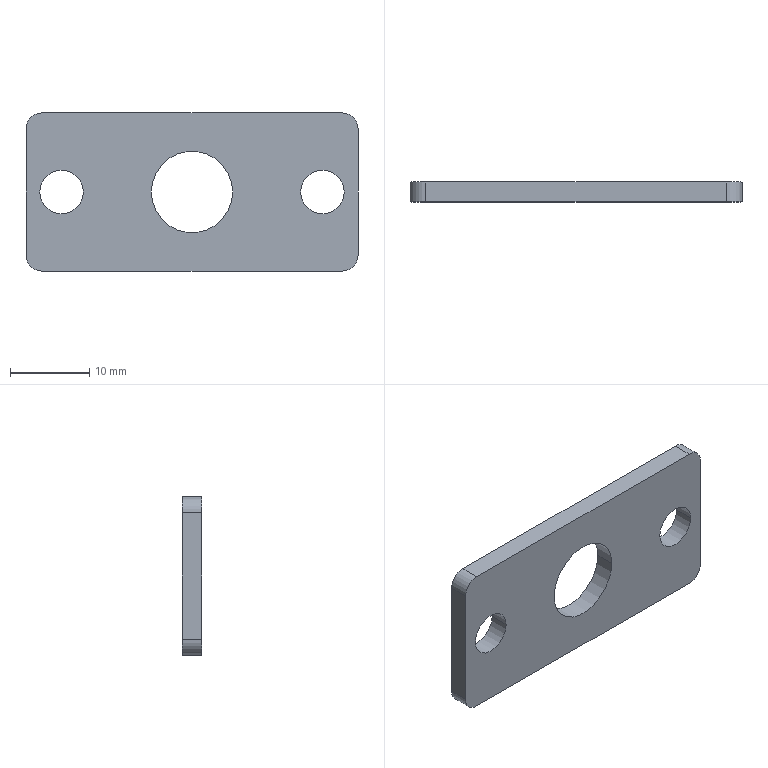Component | SolidWorks | PB_16x75_S_U_FA_M_2_0-1_F_PB12FA_16-1 | 1 solid | 16 faces | box 42 x 2.5 x 20 mm | volume 1764 mm3 | cylinder 10 | plane 6 | commonest cylinder face diameters 5.5 x4 4 x4 10.3 x2
build123d program:
from build123d import *

# Parameters (mm, degrees)
SKETCH1_R      = 2.75
SKETCH1_R_2    = 5.15
EXTRUDE1_DEPTH = 2.5


with BuildPart() as part:
    # Sketch1 → Extrude1 (new body)
    with BuildSketch(Plane.XY):
        with BuildLine():
            Line((-21, 8), (-21, -8))
            ThreePointArc((-21, -8), (-20.414, -9.414), (-19, -10))
            Line((-19, -10), (19, -10))
            ThreePointArc((19, -10), (20.414, -9.414), (21, -8))
            Line((21, -8), (21, 8))
            ThreePointArc((21, 8), (20.414, 9.414), (19, 10))
            Line((19, 10), (-19, 10))
            ThreePointArc((-19, 10), (-20.414, 9.414), (-21, 8))
        make_face()
        with Locations((16.5, 0)):
            Circle(SKETCH1_R, mode=Mode.SUBTRACT)
        Circle(SKETCH1_R_2, mode=Mode.SUBTRACT)
        with Locations((-16.5, 0)):
            Circle(SKETCH1_R, mode=Mode.SUBTRACT)
    extrude(amount=-EXTRUDE1_DEPTH)


solid = part.part

# Placed as in the assembly
solid = solid.moved(Location((45, -225, 55), (90, 0, 0)))
STEP:
#1=COLOUR_RGB('',0.7922,0.8196,0.9333);
#2=FILL_AREA_STYLE_COLOUR('',#1);
#3=FILL_AREA_STYLE('',(#2));
#4=SURFACE_STYLE_FILL_AREA(#3);
#5=SURFACE_SIDE_STYLE('',(#4));
#6=SURFACE_STYLE_USAGE(.BOTH.,#5);
#7=PRESENTATION_STYLE_ASSIGNMENT((#6));
#8=CARTESIAN_POINT('',(1.014,-8.76,2.165));
#9=VERTEX_POINT('',#8);
#10=CARTESIAN_POINT('',(1.23,-8.76,2.165));
#11=VERTEX_POINT('',#10);
#12=CARTESIAN_POINT('',(1.122,-8.76,2.165));
#13=DIRECTION('',(0.,-1.,0.));
#14=DIRECTION('',(1.,0.,0.));
#15=AXIS2_PLACEMENT_3D('',#12,#13,#14);
#16=CIRCLE('',#15,0.1083);
#17=EDGE_CURVE('',#9,#11,#16,.T.);
#18=ORIENTED_EDGE('',*,*,#17,.F.);
#19=CARTESIAN_POINT('',(1.014,-8.858,2.165));
#20=VERTEX_POINT('',#19);
#21=CARTESIAN_POINT('',(1.014,-8.76,2.165));
#22=DIRECTION('',(0.,-1.,0.));
#23=VECTOR('',#22,39.37);
#24=LINE('',#21,#23);
#25=EDGE_CURVE('',#9,#20,#24,.T.);
#26=ORIENTED_EDGE('',*,*,#25,.T.);
#27=CARTESIAN_POINT('',(1.23,-8.858,2.165));
#28=VERTEX_POINT('',#27);
#29=CARTESIAN_POINT('',(1.122,-8.858,2.165));
#30=DIRECTION('',(0.,-1.,0.));
#31=DIRECTION('',(1.,0.,0.));
#32=AXIS2_PLACEMENT_3D('',#29,#30,#31);
#33=CIRCLE('',#32,0.1083);
#34=EDGE_CURVE('',#20,#28,#33,.T.);
#35=ORIENTED_EDGE('',*,*,#34,.T.);
#36=CARTESIAN_POINT('',(1.23,-8.76,2.165));
#37=DIRECTION('',(0.,-1.,0.));
#38=VECTOR('',#37,39.37);
#39=LINE('',#36,#38);
#40=EDGE_CURVE('',#11,#28,#39,.T.);
#41=ORIENTED_EDGE('',*,*,#40,.F.);
#42=EDGE_LOOP('',(#18,#26,#35,#41));
#43=FACE_OUTER_BOUND('',#42,.T.);
#44=CARTESIAN_POINT('',(1.122,-8.76,2.165));
#45=DIRECTION('',(0.,-1.,0.));
#46=DIRECTION('',(1.,0.,0.));
#47=AXIS2_PLACEMENT_3D('',#44,#45,#46);
#48=CYLINDRICAL_SURFACE('',#47,0.1083);
#49=ADVANCED_FACE('',(#43),#48,.F.);
#50=CARTESIAN_POINT('',(1.569,-8.76,2.165));
#51=VERTEX_POINT('',#50);
#52=CARTESIAN_POINT('',(1.974,-8.76,2.165));
#53=VERTEX_POINT('',#52);
#54=CARTESIAN_POINT('',(1.772,-8.76,2.165));
#55=DIRECTION('',(0.,-1.,0.));
#56=DIRECTION('',(1.,0.,0.));
#57=AXIS2_PLACEMENT_3D('',#54,#55,#56);
#58=CIRCLE('',#57,0.2028);
#59=EDGE_CURVE('',#51,#53,#58,.T.);
#60=ORIENTED_EDGE('',*,*,#59,.F.);
#61=CARTESIAN_POINT('',(1.569,-8.858,2.165));
#62=VERTEX_POINT('',#61);
#63=CARTESIAN_POINT('',(1.569,-8.76,2.165));
#64=DIRECTION('',(0.,-1.,0.));
#65=VECTOR('',#64,39.37);
#66=LINE('',#63,#65);
#67=EDGE_CURVE('',#51,#62,#66,.T.);
#68=ORIENTED_EDGE('',*,*,#67,.T.);
#69=CARTESIAN_POINT('',(1.974,-8.858,2.165));
#70=VERTEX_POINT('',#69);
#71=CARTESIAN_POINT('',(1.772,-8.858,2.165));
#72=DIRECTION('',(0.,-1.,0.));
#73=DIRECTION('',(1.,0.,0.));
#74=AXIS2_PLACEMENT_3D('',#71,#72,#73);
#75=CIRCLE('',#74,0.2028);
#76=EDGE_CURVE('',#62,#70,#75,.T.);
#77=ORIENTED_EDGE('',*,*,#76,.T.);
#78=CARTESIAN_POINT('',(1.974,-8.76,2.165));
#79=DIRECTION('',(0.,-1.,0.));
#80=VECTOR('',#79,39.37);
#81=LINE('',#78,#80);
#82=EDGE_CURVE('',#53,#70,#81,.T.);
#83=ORIENTED_EDGE('',*,*,#82,.F.);
#84=EDGE_LOOP('',(#60,#68,#77,#83));
#85=FACE_OUTER_BOUND('',#84,.T.);
#86=CARTESIAN_POINT('',(1.772,-8.76,2.165));
#87=DIRECTION('',(0.,-1.,0.));
#88=DIRECTION('',(1.,0.,0.));
#89=AXIS2_PLACEMENT_3D('',#86,#87,#88);
#90=CYLINDRICAL_SURFACE('',#89,0.2028);
#91=ADVANCED_FACE('',(#85),#90,.F.);
#92=CARTESIAN_POINT('',(2.313,-8.76,2.165));
#93=VERTEX_POINT('',#92);
#94=CARTESIAN_POINT('',(2.53,-8.76,2.165));
#95=VERTEX_POINT('',#94);
#96=CARTESIAN_POINT('',(2.421,-8.76,2.165));
#97=DIRECTION('',(0.,-1.,0.));
#98=DIRECTION('',(1.,0.,0.));
#99=AXIS2_PLACEMENT_3D('',#96,#97,#98);
#100=CIRCLE('',#99,0.1083);
#101=EDGE_CURVE('',#93,#95,#100,.T.);
#102=ORIENTED_EDGE('',*,*,#101,.F.);
#103=CARTESIAN_POINT('',(2.313,-8.858,2.165));
#104=VERTEX_POINT('',#103);
#105=CARTESIAN_POINT('',(2.313,-8.76,2.165));
#106=DIRECTION('',(0.,-1.,0.));
#107=VECTOR('',#106,39.37);
#108=LINE('',#105,#107);
#109=EDGE_CURVE('',#93,#104,#108,.T.);
#110=ORIENTED_EDGE('',*,*,#109,.T.);
#111=CARTESIAN_POINT('',(2.53,-8.858,2.165));
#112=VERTEX_POINT('',#111);
#113=CARTESIAN_POINT('',(2.421,-8.858,2.165));
#114=DIRECTION('',(0.,-1.,0.));
#115=DIRECTION('',(1.,0.,0.));
#116=AXIS2_PLACEMENT_3D('',#113,#114,#115);
#117=CIRCLE('',#116,0.1083);
#118=EDGE_CURVE('',#104,#112,#117,.T.);
#119=ORIENTED_EDGE('',*,*,#118,.T.);
#120=CARTESIAN_POINT('',(2.53,-8.76,2.165));
#121=DIRECTION('',(0.,-1.,0.));
#122=VECTOR('',#121,39.37);
#123=LINE('',#120,#122);
#124=EDGE_CURVE('',#95,#112,#123,.T.);
#125=ORIENTED_EDGE('',*,*,#124,.F.);
#126=EDGE_LOOP('',(#102,#110,#119,#125));
#127=FACE_OUTER_BOUND('',#126,.T.);
#128=CARTESIAN_POINT('',(2.421,-8.76,2.165));
#129=DIRECTION('',(0.,-1.,0.));
#130=DIRECTION('',(1.,0.,0.));
#131=AXIS2_PLACEMENT_3D('',#128,#129,#130);
#132=CYLINDRICAL_SURFACE('',#131,0.1083);
#133=ADVANCED_FACE('',(#127),#132,.F.);
#134=CARTESIAN_POINT('',(1.024,-8.858,2.559));
#135=VERTEX_POINT('',#134);
#136=CARTESIAN_POINT('',(0.9449,-8.858,2.48));
#137=VERTEX_POINT('',#136);
#138=CARTESIAN_POINT('',(1.024,-8.858,2.48));
#139=DIRECTION('',(0.,-1.,0.));
#140=DIRECTION('',(1.,0.,0.));
#141=AXIS2_PLACEMENT_3D('',#138,#139,#140);
#142=CIRCLE('',#141,0.07874);
#143=EDGE_CURVE('',#135,#137,#142,.T.);
#144=ORIENTED_EDGE('',*,*,#143,.F.);
#145=CARTESIAN_POINT('',(1.024,-8.76,2.559));
#146=VERTEX_POINT('',#145);
#147=CARTESIAN_POINT('',(1.024,-8.76,2.559));
#148=DIRECTION('',(0.,-1.,0.));
#149=VECTOR('',#148,39.37);
#150=LINE('',#147,#149);
#151=EDGE_CURVE('',#146,#135,#150,.T.);
#152=ORIENTED_EDGE('',*,*,#151,.F.);
#153=CARTESIAN_POINT('',(0.9449,-8.76,2.48));
#154=VERTEX_POINT('',#153);
#155=CARTESIAN_POINT('',(1.024,-8.76,2.48));
#156=DIRECTION('',(0.,-1.,0.));
#157=DIRECTION('',(1.,0.,0.));
#158=AXIS2_PLACEMENT_3D('',#155,#156,#157);
#159=CIRCLE('',#158,0.07874);
#160=EDGE_CURVE('',#146,#154,#159,.T.);
#161=ORIENTED_EDGE('',*,*,#160,.T.);
#162=CARTESIAN_POINT('',(0.9449,-8.76,2.48));
#163=DIRECTION('',(0.,-1.,0.));
#164=VECTOR('',#163,39.37);
#165=LINE('',#162,#164);
#166=EDGE_CURVE('',#154,#137,#165,.T.);
#167=ORIENTED_EDGE('',*,*,#166,.T.);
#168=EDGE_LOOP('',(#144,#152,#161,#167));
#169=FACE_OUTER_BOUND('',#168,.T.);
#170=CARTESIAN_POINT('',(1.024,-8.76,2.48));
#171=DIRECTION('',(0.,-1.,0.));
#172=DIRECTION('',(1.,0.,0.));
#173=AXIS2_PLACEMENT_3D('',#170,#171,#172);
#174=CYLINDRICAL_SURFACE('',#173,0.07874);
#175=ADVANCED_FACE('',(#169),#174,.T.);
#176=CARTESIAN_POINT('',(2.52,-8.858,2.559));
#177=VERTEX_POINT('',#176);
#178=CARTESIAN_POINT('',(2.52,-8.858,2.559));
#179=DIRECTION('',(-1.,0.,0.));
#180=VECTOR('',#179,39.37);
#181=LINE('',#178,#180);
#182=EDGE_CURVE('',#177,#135,#181,.T.);
#183=ORIENTED_EDGE('',*,*,#182,.F.);
#184=CARTESIAN_POINT('',(2.52,-8.76,2.559));
#185=VERTEX_POINT('',#184);
#186=CARTESIAN_POINT('',(2.52,-8.76,2.559));
#187=DIRECTION('',(0.,-1.,0.));
#188=VECTOR('',#187,39.37);
#189=LINE('',#186,#188);
#190=EDGE_CURVE('',#185,#177,#189,.T.);
#191=ORIENTED_EDGE('',*,*,#190,.F.);
#192=CARTESIAN_POINT('',(2.52,-8.76,2.559));
#193=DIRECTION('',(-1.,0.,0.));
#194=VECTOR('',#193,39.37);
#195=LINE('',#192,#194);
#196=EDGE_CURVE('',#185,#146,#195,.T.);
#197=ORIENTED_EDGE('',*,*,#196,.T.);
#198=ORIENTED_EDGE('',*,*,#151,.T.);
#199=EDGE_LOOP('',(#183,#191,#197,#198));
#200=FACE_OUTER_BOUND('',#199,.T.);
#201=CARTESIAN_POINT('',(2.52,-8.76,2.559));
#202=DIRECTION('',(0.,0.,1.));
#203=DIRECTION('',(0.,-1.,0.));
#204=AXIS2_PLACEMENT_3D('',#201,#202,#203);
#205=PLANE('',#204);
#206=ADVANCED_FACE('',(#200),#205,.T.);
#207=CARTESIAN_POINT('',(2.598,-8.858,2.48));
#208=VERTEX_POINT('',#207);
#209=CARTESIAN_POINT('',(2.52,-8.858,2.48));
#210=DIRECTION('',(0.,-1.,0.));
#211=DIRECTION('',(1.,0.,0.));
#212=AXIS2_PLACEMENT_3D('',#209,#210,#211);
#213=CIRCLE('',#212,0.07874);
#214=EDGE_CURVE('',#208,#177,#213,.T.);
#215=ORIENTED_EDGE('',*,*,#214,.F.);
#216=CARTESIAN_POINT('',(2.598,-8.76,2.48));
#217=VERTEX_POINT('',#216);
#218=CARTESIAN_POINT('',(2.598,-8.76,2.48));
#219=DIRECTION('',(0.,-1.,0.));
#220=VECTOR('',#219,39.37);
#221=LINE('',#218,#220);
#222=EDGE_CURVE('',#217,#208,#221,.T.);
#223=ORIENTED_EDGE('',*,*,#222,.F.);
#224=CARTESIAN_POINT('',(2.52,-8.76,2.48));
#225=DIRECTION('',(0.,-1.,0.));
#226=DIRECTION('',(1.,0.,0.));
#227=AXIS2_PLACEMENT_3D('',#224,#225,#226);
#228=CIRCLE('',#227,0.07874);
#229=EDGE_CURVE('',#217,#185,#228,.T.);
#230=ORIENTED_EDGE('',*,*,#229,.T.);
#231=ORIENTED_EDGE('',*,*,#190,.T.);
#232=EDGE_LOOP('',(#215,#223,#230,#231));
#233=FACE_OUTER_BOUND('',#232,.T.);
#234=CARTESIAN_POINT('',(2.52,-8.76,2.48));
#235=DIRECTION('',(0.,-1.,0.));
#236=DIRECTION('',(1.,0.,0.));
#237=AXIS2_PLACEMENT_3D('',#234,#235,#236);
#238=CYLINDRICAL_SURFACE('',#237,0.07874);
#239=ADVANCED_FACE('',(#233),#238,.T.);
#240=CARTESIAN_POINT('',(2.598,-8.858,1.85));
#241=VERTEX_POINT('',#240);
#242=CARTESIAN_POINT('',(2.598,-8.858,1.85));
#243=DIRECTION('',(0.,0.,1.));
#244=VECTOR('',#243,39.37);
#245=LINE('',#242,#244);
#246=EDGE_CURVE('',#241,#208,#245,.T.);
#247=ORIENTED_EDGE('',*,*,#246,.F.);
#248=CARTESIAN_POINT('',(2.598,-8.76,1.85));
#249=VERTEX_POINT('',#248);
#250=CARTESIAN_POINT('',(2.598,-8.76,1.85));
#251=DIRECTION('',(0.,-1.,0.));
#252=VECTOR('',#251,39.37);
#253=LINE('',#250,#252);
#254=EDGE_CURVE('',#249,#241,#253,.T.);
#255=ORIENTED_EDGE('',*,*,#254,.F.);
#256=CARTESIAN_POINT('',(2.598,-8.76,1.85));
#257=DIRECTION('',(0.,0.,1.));
#258=VECTOR('',#257,39.37);
#259=LINE('',#256,#258);
#260=EDGE_CURVE('',#249,#217,#259,.T.);
#261=ORIENTED_EDGE('',*,*,#260,.T.);
#262=ORIENTED_EDGE('',*,*,#222,.T.);
#263=EDGE_LOOP('',(#247,#255,#261,#262));
#264=FACE_OUTER_BOUND('',#263,.T.);
#265=CARTESIAN_POINT('',(2.598,-8.76,1.85));
#266=DIRECTION('',(1.,0.,0.));
#267=DIRECTION('',(0.,1.,0.));
#268=AXIS2_PLACEMENT_3D('',#265,#266,#267);
#269=PLANE('',#268);
#270=ADVANCED_FACE('',(#264),#269,.T.);
#271=CARTESIAN_POINT('',(2.52,-8.858,1.772));
#272=VERTEX_POINT('',#271);
#273=CARTESIAN_POINT('',(2.52,-8.858,1.85));
#274=DIRECTION('',(0.,-1.,0.));
#275=DIRECTION('',(1.,0.,0.));
#276=AXIS2_PLACEMENT_3D('',#273,#274,#275);
#277=CIRCLE('',#276,0.07874);
#278=EDGE_CURVE('',#272,#241,#277,.T.);
#279=ORIENTED_EDGE('',*,*,#278,.F.);
#280=CARTESIAN_POINT('',(2.52,-8.76,1.772));
#281=VERTEX_POINT('',#280);
#282=CARTESIAN_POINT('',(2.52,-8.76,1.772));
#283=DIRECTION('',(0.,-1.,0.));
#284=VECTOR('',#283,39.37);
#285=LINE('',#282,#284);
#286=EDGE_CURVE('',#281,#272,#285,.T.);
#287=ORIENTED_EDGE('',*,*,#286,.F.);
#288=CARTESIAN_POINT('',(2.52,-8.76,1.85));
#289=DIRECTION('',(0.,-1.,0.));
#290=DIRECTION('',(1.,0.,0.));
#291=AXIS2_PLACEMENT_3D('',#288,#289,#290);
#292=CIRCLE('',#291,0.07874);
#293=EDGE_CURVE('',#281,#249,#292,.T.);
#294=ORIENTED_EDGE('',*,*,#293,.T.);
#295=ORIENTED_EDGE('',*,*,#254,.T.);
#296=EDGE_LOOP('',(#279,#287,#294,#295));
#297=FACE_OUTER_BOUND('',#296,.T.);
#298=CARTESIAN_POINT('',(2.52,-8.76,1.85));
#299=DIRECTION('',(0.,-1.,0.));
#300=DIRECTION('',(1.,0.,0.));
#301=AXIS2_PLACEMENT_3D('',#298,#299,#300);
#302=CYLINDRICAL_SURFACE('',#301,0.07874);
#303=ADVANCED_FACE('',(#297),#302,.T.);
#304=CARTESIAN_POINT('',(1.024,-8.858,1.772));
#305=VERTEX_POINT('',#304);
#306=CARTESIAN_POINT('',(1.024,-8.858,1.772));
#307=DIRECTION('',(1.,0.,0.));
#308=VECTOR('',#307,39.37);
#309=LINE('',#306,#308);
#310=EDGE_CURVE('',#305,#272,#309,.T.);
#311=ORIENTED_EDGE('',*,*,#310,.F.);
#312=CARTESIAN_POINT('',(1.024,-8.76,1.772));
#313=VERTEX_POINT('',#312);
#314=CARTESIAN_POINT('',(1.024,-8.76,1.772));
#315=DIRECTION('',(0.,-1.,0.));
#316=VECTOR('',#315,39.37);
#317=LINE('',#314,#316);
#318=EDGE_CURVE('',#313,#305,#317,.T.);
#319=ORIENTED_EDGE('',*,*,#318,.F.);
#320=CARTESIAN_POINT('',(1.024,-8.76,1.772));
#321=DIRECTION('',(1.,0.,0.));
#322=VECTOR('',#321,39.37);
#323=LINE('',#320,#322);
#324=EDGE_CURVE('',#313,#281,#323,.T.);
#325=ORIENTED_EDGE('',*,*,#324,.T.);
#326=ORIENTED_EDGE('',*,*,#286,.T.);
#327=EDGE_LOOP('',(#311,#319,#325,#326));
#328=FACE_OUTER_BOUND('',#327,.T.);
#329=CARTESIAN_POINT('',(1.024,-8.76,1.772));
#330=DIRECTION('',(0.,0.,-1.));
#331=DIRECTION('',(0.,1.,0.));
#332=AXIS2_PLACEMENT_3D('',#329,#330,#331);
#333=PLANE('',#332);
#334=ADVANCED_FACE('',(#328),#333,.T.);
#335=CARTESIAN_POINT('',(0.9449,-8.858,1.85));
#336=VERTEX_POINT('',#335);
#337=CARTESIAN_POINT('',(1.024,-8.858,1.85));
#338=DIRECTION('',(0.,-1.,0.));
#339=DIRECTION('',(1.,0.,0.));
#340=AXIS2_PLACEMENT_3D('',#337,#338,#339);
#341=CIRCLE('',#340,0.07874);
#342=EDGE_CURVE('',#336,#305,#341,.T.);
#343=ORIENTED_EDGE('',*,*,#342,.F.);
#344=CARTESIAN_POINT('',(0.9449,-8.76,1.85));
#345=VERTEX_POINT('',#344);
#346=CARTESIAN_POINT('',(0.9449,-8.76,1.85));
#347=DIRECTION('',(0.,-1.,0.));
#348=VECTOR('',#347,39.37);
#349=LINE('',#346,#348);
#350=EDGE_CURVE('',#345,#336,#349,.T.);
#351=ORIENTED_EDGE('',*,*,#350,.F.);
#352=CARTESIAN_POINT('',(1.024,-8.76,1.85));
#353=DIRECTION('',(0.,-1.,0.));
#354=DIRECTION('',(1.,0.,0.));
#355=AXIS2_PLACEMENT_3D('',#352,#353,#354);
#356=CIRCLE('',#355,0.07874);
#357=EDGE_CURVE('',#345,#313,#356,.T.);
#358=ORIENTED_EDGE('',*,*,#357,.T.);
#359=ORIENTED_EDGE('',*,*,#318,.T.);
#360=EDGE_LOOP('',(#343,#351,#358,#359));
#361=FACE_OUTER_BOUND('',#360,.T.);
#362=CARTESIAN_POINT('',(1.024,-8.76,1.85));
#363=DIRECTION('',(0.,-1.,0.));
#364=DIRECTION('',(1.,0.,0.));
#365=AXIS2_PLACEMENT_3D('',#362,#363,#364);
#366=CYLINDRICAL_SURFACE('',#365,0.07874);
#367=ADVANCED_FACE('',(#361),#366,.T.);
#368=CARTESIAN_POINT('',(0.9449,-8.858,2.48));
#369=DIRECTION('',(0.,0.,-1.));
#370=VECTOR('',#369,39.37);
#371=LINE('',#368,#370);
#372=EDGE_CURVE('',#137,#336,#371,.T.);
#373=ORIENTED_EDGE('',*,*,#372,.F.);
#374=ORIENTED_EDGE('',*,*,#166,.F.);
#375=CARTESIAN_POINT('',(0.9449,-8.76,2.48));
#376=DIRECTION('',(0.,0.,-1.));
#377=VECTOR('',#376,39.37);
#378=LINE('',#375,#377);
#379=EDGE_CURVE('',#154,#345,#378,.T.);
#380=ORIENTED_EDGE('',*,*,#379,.T.);
#381=ORIENTED_EDGE('',*,*,#350,.T.);
#382=EDGE_LOOP('',(#373,#374,#380,#381));
#383=FACE_OUTER_BOUND('',#382,.T.);
#384=CARTESIAN_POINT('',(0.9449,-8.76,2.48));
#385=DIRECTION('',(-1.,0.,0.));
#386=DIRECTION('',(0.,-1.,0.));
#387=AXIS2_PLACEMENT_3D('',#384,#385,#386);
#388=PLANE('',#387);
#389=ADVANCED_FACE('',(#383),#388,.T.);
#390=CARTESIAN_POINT('',(1.122,-8.76,2.165));
#391=DIRECTION('',(0.,-1.,0.));
#392=DIRECTION('',(1.,0.,0.));
#393=AXIS2_PLACEMENT_3D('',#390,#391,#392);
#394=CIRCLE('',#393,0.1083);
#395=EDGE_CURVE('',#11,#9,#394,.T.);
#396=ORIENTED_EDGE('',*,*,#395,.T.);
#397=ORIENTED_EDGE('',*,*,#17,.T.);
#398=EDGE_LOOP('',(#396,#397));
#399=FACE_BOUND('',#398,.T.);
#400=CARTESIAN_POINT('',(1.772,-8.76,2.165));
#401=DIRECTION('',(0.,-1.,0.));
#402=DIRECTION('',(1.,0.,0.));
#403=AXIS2_PLACEMENT_3D('',#400,#401,#402);
#404=CIRCLE('',#403,0.2028);
#405=EDGE_CURVE('',#53,#51,#404,.T.);
#406=ORIENTED_EDGE('',*,*,#405,.T.);
#407=ORIENTED_EDGE('',*,*,#59,.T.);
#408=EDGE_LOOP('',(#406,#407));
#409=FACE_BOUND('',#408,.T.);
#410=CARTESIAN_POINT('',(2.421,-8.76,2.165));
#411=DIRECTION('',(0.,-1.,0.));
#412=DIRECTION('',(1.,0.,0.));
#413=AXIS2_PLACEMENT_3D('',#410,#411,#412);
#414=CIRCLE('',#413,0.1083);
#415=EDGE_CURVE('',#95,#93,#414,.T.);
#416=ORIENTED_EDGE('',*,*,#415,.T.);
#417=ORIENTED_EDGE('',*,*,#101,.T.);
#418=EDGE_LOOP('',(#416,#417));
#419=FACE_BOUND('',#418,.T.);
#420=ORIENTED_EDGE('',*,*,#160,.F.);
#421=ORIENTED_EDGE('',*,*,#196,.F.);
#422=ORIENTED_EDGE('',*,*,#229,.F.);
#423=ORIENTED_EDGE('',*,*,#260,.F.);
#424=ORIENTED_EDGE('',*,*,#293,.F.);
#425=ORIENTED_EDGE('',*,*,#324,.F.);
#426=ORIENTED_EDGE('',*,*,#357,.F.);
#427=ORIENTED_EDGE('',*,*,#379,.F.);
#428=EDGE_LOOP('',(#420,#421,#422,#423,#424,#425,#426,#427));
#429=FACE_OUTER_BOUND('',#428,.T.);
#430=CARTESIAN_POINT('',(1.024,-8.76,2.48));
#431=DIRECTION('',(0.,-1.,0.));
#432=DIRECTION('',(1.,0.,0.));
#433=AXIS2_PLACEMENT_3D('',#430,#431,#432);
#434=PLANE('',#433);
#435=ADVANCED_FACE('',(#399,#409,#419,#429),#434,.F.);
#436=CARTESIAN_POINT('',(1.122,-8.858,2.165));
#437=DIRECTION('',(0.,-1.,0.));
#438=DIRECTION('',(1.,0.,0.));
#439=AXIS2_PLACEMENT_3D('',#436,#437,#438);
#440=CIRCLE('',#439,0.1083);
#441=EDGE_CURVE('',#28,#20,#440,.T.);
#442=ORIENTED_EDGE('',*,*,#441,.F.);
#443=ORIENTED_EDGE('',*,*,#34,.F.);
#444=EDGE_LOOP('',(#442,#443));
#445=FACE_BOUND('',#444,.T.);
#446=CARTESIAN_POINT('',(1.772,-8.858,2.165));
#447=DIRECTION('',(0.,-1.,0.));
#448=DIRECTION('',(1.,0.,0.));
#449=AXIS2_PLACEMENT_3D('',#446,#447,#448);
#450=CIRCLE('',#449,0.2028);
#451=EDGE_CURVE('',#70,#62,#450,.T.);
#452=ORIENTED_EDGE('',*,*,#451,.F.);
#453=ORIENTED_EDGE('',*,*,#76,.F.);
#454=EDGE_LOOP('',(#452,#453));
#455=FACE_BOUND('',#454,.T.);
#456=CARTESIAN_POINT('',(2.421,-8.858,2.165));
#457=DIRECTION('',(0.,-1.,0.));
#458=DIRECTION('',(1.,0.,0.));
#459=AXIS2_PLACEMENT_3D('',#456,#457,#458);
#460=CIRCLE('',#459,0.1083);
#461=EDGE_CURVE('',#112,#104,#460,.T.);
#462=ORIENTED_EDGE('',*,*,#461,.F.);
#463=ORIENTED_EDGE('',*,*,#118,.F.);
#464=EDGE_LOOP('',(#462,#463));
#465=FACE_BOUND('',#464,.T.);
#466=ORIENTED_EDGE('',*,*,#143,.T.);
#467=ORIENTED_EDGE('',*,*,#372,.T.);
#468=ORIENTED_EDGE('',*,*,#342,.T.);
#469=ORIENTED_EDGE('',*,*,#310,.T.);
#470=ORIENTED_EDGE('',*,*,#278,.T.);
#471=ORIENTED_EDGE('',*,*,#246,.T.);
#472=ORIENTED_EDGE('',*,*,#214,.T.);
#473=ORIENTED_EDGE('',*,*,#182,.T.);
#474=EDGE_LOOP('',(#466,#467,#468,#469,#470,#471,#472,#473));
#475=FACE_OUTER_BOUND('',#474,.T.);
#476=CARTESIAN_POINT('',(1.024,-8.858,2.48));
#477=DIRECTION('',(0.,-1.,0.));
#478=DIRECTION('',(1.,0.,0.));
#479=AXIS2_PLACEMENT_3D('',#476,#477,#478);
#480=PLANE('',#479);
#481=ADVANCED_FACE('',(#445,#455,#465,#475),#480,.T.);
#482=ORIENTED_EDGE('',*,*,#109,.F.);
#483=ORIENTED_EDGE('',*,*,#415,.F.);
#484=ORIENTED_EDGE('',*,*,#124,.T.);
#485=ORIENTED_EDGE('',*,*,#461,.T.);
#486=EDGE_LOOP('',(#482,#483,#484,#485));
#487=FACE_OUTER_BOUND('',#486,.T.);
#488=CARTESIAN_POINT('',(2.421,-8.76,2.165));
#489=DIRECTION('',(0.,-1.,0.));
#490=DIRECTION('',(1.,0.,0.));
#491=AXIS2_PLACEMENT_3D('',#488,#489,#490);
#492=CYLINDRICAL_SURFACE('',#491,0.1083);
#493=ADVANCED_FACE('',(#487),#492,.F.);
#494=ORIENTED_EDGE('',*,*,#67,.F.);
#495=ORIENTED_EDGE('',*,*,#405,.F.);
#496=ORIENTED_EDGE('',*,*,#82,.T.);
#497=ORIENTED_EDGE('',*,*,#451,.T.);
#498=EDGE_LOOP('',(#494,#495,#496,#497));
#499=FACE_OUTER_BOUND('',#498,.T.);
#500=CARTESIAN_POINT('',(1.772,-8.76,2.165));
#501=DIRECTION('',(0.,-1.,0.));
#502=DIRECTION('',(1.,0.,0.));
#503=AXIS2_PLACEMENT_3D('',#500,#501,#502);
#504=CYLINDRICAL_SURFACE('',#503,0.2028);
#505=ADVANCED_FACE('',(#499),#504,.F.);
#506=ORIENTED_EDGE('',*,*,#25,.F.);
#507=ORIENTED_EDGE('',*,*,#395,.F.);
#508=ORIENTED_EDGE('',*,*,#40,.T.);
#509=ORIENTED_EDGE('',*,*,#441,.T.);
#510=EDGE_LOOP('',(#506,#507,#508,#509));
#511=FACE_OUTER_BOUND('',#510,.T.);
#512=CARTESIAN_POINT('',(1.122,-8.76,2.165));
#513=DIRECTION('',(0.,-1.,0.));
#514=DIRECTION('',(1.,0.,0.));
#515=AXIS2_PLACEMENT_3D('',#512,#513,#514);
#516=CYLINDRICAL_SURFACE('',#515,0.1083);
#517=ADVANCED_FACE('',(#511),#516,.F.);
#518=CLOSED_SHELL('',(#49,#91,#133,#175,#206,#239,#270,#303,#334,#367,#389,#435,#481,#493,#505,#517));
#519=MANIFOLD_SOLID_BREP('',#518);
#520=STYLED_ITEM('',(#7),#519);
#521=PRESENTATION_LAYER_ASSIGNMENT('','',(#520));
#522=(LENGTH_UNIT()NAMED_UNIT(*)SI_UNIT($,.METRE.));
#523=LENGTH_MEASURE_WITH_UNIT(LENGTH_MEASURE(0.0254),#522);
#524=DIMENSIONAL_EXPONENTS(1.,0.,0.,0.,0.,0.,0.);
#525=(CONVERSION_BASED_UNIT('',#523)LENGTH_UNIT()NAMED_UNIT(#524));
#526=UNCERTAINTY_MEASURE_WITH_UNIT(LENGTH_MEASURE(0.00001),#525,'','');
#527=(NAMED_UNIT(*)PLANE_ANGLE_UNIT()SI_UNIT($,.RADIAN.));
#528=(NAMED_UNIT(*)SI_UNIT($,.STERADIAN.)SOLID_ANGLE_UNIT());
#529=(GEOMETRIC_REPRESENTATION_CONTEXT(3)GLOBAL_UNCERTAINTY_ASSIGNED_CONTEXT((#526))GLOBAL_UNIT_ASSIGNED_CONTEXT((#525,#527,#528))REPRESENTATION_CONTEXT('',''));
#530=MECHANICAL_DESIGN_GEOMETRIC_PRESENTATION_REPRESENTATION('',(#520),#529);
#531=CARTESIAN_POINT('',(0.,0.,0.));
#532=DIRECTION('',(0.,0.,1.));
#533=DIRECTION('',(1.,0.,0.));
#534=AXIS2_PLACEMENT_3D('',#531,#532,#533);
#535=(LENGTH_UNIT()NAMED_UNIT(*)SI_UNIT($,.METRE.));
#536=LENGTH_MEASURE_WITH_UNIT(LENGTH_MEASURE(0.0254),#535);
#537=DIMENSIONAL_EXPONENTS(1.,0.,0.,0.,0.,0.,0.);
#538=(CONVERSION_BASED_UNIT('',#536)LENGTH_UNIT()NAMED_UNIT(#537));
#539=UNCERTAINTY_MEASURE_WITH_UNIT(LENGTH_MEASURE(0.00001),#538,'','');
#540=(NAMED_UNIT(*)PLANE_ANGLE_UNIT()SI_UNIT($,.RADIAN.));
#541=(NAMED_UNIT(*)SI_UNIT($,.STERADIAN.)SOLID_ANGLE_UNIT());
#542=(GEOMETRIC_REPRESENTATION_CONTEXT(3)GLOBAL_UNCERTAINTY_ASSIGNED_CONTEXT((#539))GLOBAL_UNIT_ASSIGNED_CONTEXT((#538,#540,#541))REPRESENTATION_CONTEXT('',''));
#543=ADVANCED_BREP_SHAPE_REPRESENTATION('',(#519,#534),#542);